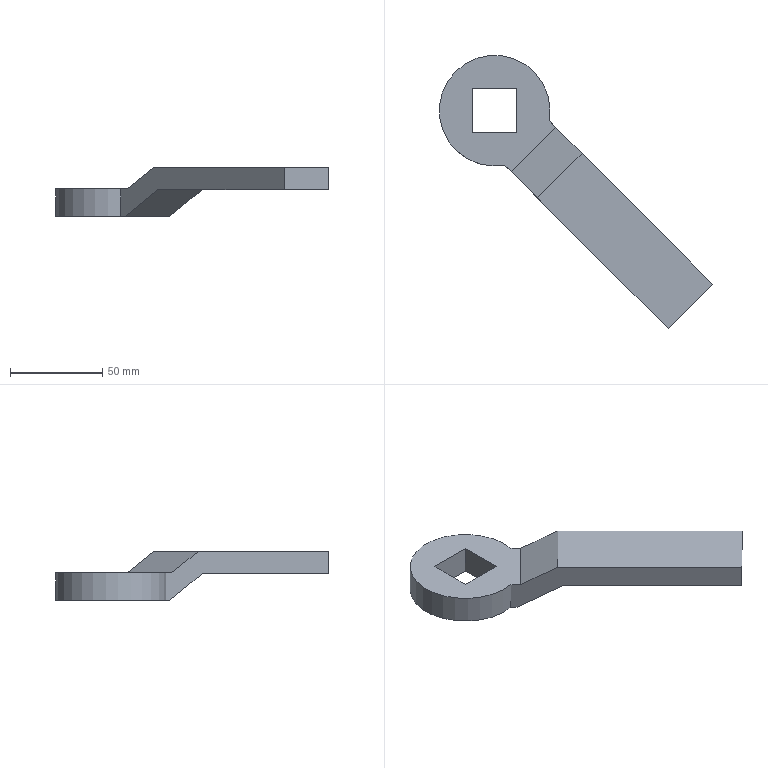Component | NX | WRENCH | 1 solid | 14 faces | box 148.09 x 148.09 x 26.55 mm | volume 84920 mm3 | plane 13 | cylinder 1 | commonest cylinder face diameters 60 x1
STEP:
#1=CARTESIAN_POINT('',(0.,0.,0.));
#2=DIRECTION('',(0.,0.,1.));
#3=DIRECTION('',(1.,0.,0.));
#4=AXIS2_PLACEMENT_3D('',#1,#2,#3);
#5=CARTESIAN_POINT('',(1.86,-30.695,193.134));
#6=VERTEX_POINT('',#5);
#7=CARTESIAN_POINT('',(25.901,-6.653,193.134));
#8=VERTEX_POINT('',#7);
#9=CARTESIAN_POINT('',(1.86,-30.695,193.134));
#10=DIRECTION('',(0.7071,0.7071,0.));
#11=VECTOR('',#10,1.);
#12=LINE('',#9,#11);
#13=CARTESIAN_POINT('',(1.86,-30.695,193.134));
#14=DIRECTION('',(-0.3536,0.3536,0.866));
#15=DIRECTION('',(0.6124,-0.6124,0.5));
#16=AXIS2_PLACEMENT_3D('',#13,#14,#15);
#17=PLANE('',#16);
#18=CARTESIAN_POINT('',(0.,0.));
#19=DIRECTION('',(-0.,1.));
#20=VECTOR('',#19,1.);
#21=LINE('',#18,#20);
#22=(GEOMETRIC_REPRESENTATION_CONTEXT(2)PARAMETRIC_REPRESENTATION_CONTEXT()REPRESENTATION_CONTEXT('',''));
#23=DEFINITIONAL_REPRESENTATION('',(#21),#22);
#24=PCURVE('',#17,#23);
#25=CARTESIAN_POINT('',(-5.932,1.139,193.134));
#26=DIRECTION('',(0.,0.,-1.));
#27=DIRECTION('',(-0.7071,0.7071,0.));
#28=AXIS2_PLACEMENT_3D('',#25,#26,#27);
#29=PLANE('',#28);
#30=CARTESIAN_POINT('',(-28.019,-17.));
#31=DIRECTION('',(0.,1.));
#32=VECTOR('',#31,1.);
#33=LINE('',#30,#32);
#34=(GEOMETRIC_REPRESENTATION_CONTEXT(2)PARAMETRIC_REPRESENTATION_CONTEXT()REPRESENTATION_CONTEXT('',''));
#35=DEFINITIONAL_REPRESENTATION('',(#33),#34);
#36=PCURVE('',#29,#35);
#37=SURFACE_CURVE('',#12,(#24,#36),.PCURVE_S1.);
#38=EDGE_CURVE('',#6,#8,#37,.T.);
#39=ORIENTED_EDGE('',*,*,#38,.T.);
#40=CARTESIAN_POINT('',(43.718,-24.469,207.681));
#41=VERTEX_POINT('',#40);
#42=CARTESIAN_POINT('',(25.901,-6.653,193.134));
#43=DIRECTION('',(0.6124,-0.6124,0.5));
#44=VECTOR('',#43,1.);
#45=LINE('',#42,#44);
#46=CARTESIAN_POINT('',(-0.,34.));
#47=DIRECTION('',(1.,0.));
#48=VECTOR('',#47,1.);
#49=LINE('',#46,#48);
#50=(GEOMETRIC_REPRESENTATION_CONTEXT(2)PARAMETRIC_REPRESENTATION_CONTEXT()REPRESENTATION_CONTEXT('',''));
#51=DEFINITIONAL_REPRESENTATION('',(#49),#50);
#52=PCURVE('',#17,#51);
#53=CARTESIAN_POINT('',(6.089,13.16,193.134));
#54=DIRECTION('',(-0.7071,-0.7071,0.));
#55=DIRECTION('',(0.,0.,-1.));
#56=AXIS2_PLACEMENT_3D('',#53,#54,#55);
#57=PLANE('',#56);
#58=CARTESIAN_POINT('',(0.,28.019));
#59=DIRECTION('',(-0.5,0.866));
#60=VECTOR('',#59,1.);
#61=LINE('',#58,#60);
#62=(GEOMETRIC_REPRESENTATION_CONTEXT(2)PARAMETRIC_REPRESENTATION_CONTEXT()REPRESENTATION_CONTEXT('',''));
#63=DEFINITIONAL_REPRESENTATION('',(#61),#62);
#64=PCURVE('',#57,#63);
#65=SURFACE_CURVE('',#45,(#52,#64),.PCURVE_S1.);
#66=EDGE_CURVE('',#8,#41,#65,.T.);
#67=ORIENTED_EDGE('',*,*,#66,.T.);
#68=CARTESIAN_POINT('',(19.676,-48.511,207.681));
#69=VERTEX_POINT('',#68);
#70=CARTESIAN_POINT('',(19.676,-48.511,207.681));
#71=DIRECTION('',(0.7071,0.7071,0.));
#72=VECTOR('',#71,1.);
#73=LINE('',#70,#72);
#74=CARTESIAN_POINT('',(29.094,0.));
#75=DIRECTION('',(-0.,1.));
#76=VECTOR('',#75,1.);
#77=LINE('',#74,#76);
#78=(GEOMETRIC_REPRESENTATION_CONTEXT(2)PARAMETRIC_REPRESENTATION_CONTEXT()REPRESENTATION_CONTEXT('',''));
#79=DEFINITIONAL_REPRESENTATION('',(#77),#78);
#80=PCURVE('',#17,#79);
#81=CARTESIAN_POINT('',(19.676,-48.511,207.681));
#82=DIRECTION('',(0.,0.,1.));
#83=DIRECTION('',(0.7071,-0.7071,0.));
#84=AXIS2_PLACEMENT_3D('',#81,#82,#83);
#85=PLANE('',#84);
#86=CARTESIAN_POINT('',(0.,0.));
#87=DIRECTION('',(0.,1.));
#88=VECTOR('',#87,1.);
#89=LINE('',#86,#88);
#90=(GEOMETRIC_REPRESENTATION_CONTEXT(2)PARAMETRIC_REPRESENTATION_CONTEXT()REPRESENTATION_CONTEXT('',''));
#91=DEFINITIONAL_REPRESENTATION('',(#89),#90);
#92=PCURVE('',#85,#91);
#93=SURFACE_CURVE('',#73,(#80,#92),.PCURVE_S1.);
#94=EDGE_CURVE('',#69,#41,#93,.T.);
#95=ORIENTED_EDGE('',*,*,#94,.F.);
#96=CARTESIAN_POINT('',(1.86,-30.695,193.134));
#97=DIRECTION('',(0.6124,-0.6124,0.5));
#98=VECTOR('',#97,1.);
#99=LINE('',#96,#98);
#100=CARTESIAN_POINT('',(0.,0.));
#101=DIRECTION('',(1.,0.));
#102=VECTOR('',#101,1.);
#103=LINE('',#100,#102);
#104=(GEOMETRIC_REPRESENTATION_CONTEXT(2)PARAMETRIC_REPRESENTATION_CONTEXT()REPRESENTATION_CONTEXT('',''));
#105=DEFINITIONAL_REPRESENTATION('',(#103),#104);
#106=PCURVE('',#17,#105);
#107=CARTESIAN_POINT('',(-17.953,-10.882,193.134));
#108=DIRECTION('',(-0.7071,-0.7071,0.));
#109=DIRECTION('',(0.,0.,-1.));
#110=AXIS2_PLACEMENT_3D('',#107,#108,#109);
#111=PLANE('',#110);
#112=CARTESIAN_POINT('',(0.,28.019));
#113=DIRECTION('',(-0.5,0.866));
#114=VECTOR('',#113,1.);
#115=LINE('',#112,#114);
#116=(GEOMETRIC_REPRESENTATION_CONTEXT(2)PARAMETRIC_REPRESENTATION_CONTEXT()REPRESENTATION_CONTEXT('',''));
#117=DEFINITIONAL_REPRESENTATION('',(#115),#116);
#118=PCURVE('',#111,#117);
#119=SURFACE_CURVE('',#99,(#106,#118),.PCURVE_S1.);
#120=EDGE_CURVE('',#6,#69,#119,.T.);
#121=ORIENTED_EDGE('',*,*,#120,.F.);
#122=EDGE_LOOP('',(#39,#67,#95,#121));
#123=FACE_BOUND('',#122,.T.);
#124=ADVANCED_FACE('',(#123),#17,.F.);
#125=CARTESIAN_POINT('',(-17.932,13.139,208.134));
#126=VERTEX_POINT('',#125);
#127=CARTESIAN_POINT('',(-17.932,-10.861,208.134));
#128=VERTEX_POINT('',#127);
#129=CARTESIAN_POINT('',(-17.932,13.139,208.134));
#130=DIRECTION('',(0.,-1.,0.));
#131=VECTOR('',#130,1.);
#132=LINE('',#129,#131);
#133=CARTESIAN_POINT('',(-5.932,1.139,208.134));
#134=DIRECTION('',(0.,0.,1.));
#135=DIRECTION('',(0.7071,-0.7071,0.));
#136=AXIS2_PLACEMENT_3D('',#133,#134,#135);
#137=PLANE('',#136);
#138=CARTESIAN_POINT('',(-16.971,0.));
#139=DIRECTION('',(0.7071,-0.7071));
#140=VECTOR('',#139,1.);
#141=LINE('',#138,#140);
#142=(GEOMETRIC_REPRESENTATION_CONTEXT(2)PARAMETRIC_REPRESENTATION_CONTEXT()REPRESENTATION_CONTEXT('',''));
#143=DEFINITIONAL_REPRESENTATION('',(#141),#142);
#144=PCURVE('',#137,#143);
#145=CARTESIAN_POINT('',(-17.932,13.139,191.134));
#146=DIRECTION('',(-1.,0.,0.));
#147=DIRECTION('',(0.,-1.,0.));
#148=AXIS2_PLACEMENT_3D('',#145,#146,#147);
#149=PLANE('',#148);
#150=CARTESIAN_POINT('',(0.,17.));
#151=DIRECTION('',(1.,0.));
#152=VECTOR('',#151,1.);
#153=LINE('',#150,#152);
#154=(GEOMETRIC_REPRESENTATION_CONTEXT(2)PARAMETRIC_REPRESENTATION_CONTEXT()REPRESENTATION_CONTEXT('',''));
#155=DEFINITIONAL_REPRESENTATION('',(#153),#154);
#156=PCURVE('',#149,#155);
#157=SURFACE_CURVE('',#132,(#144,#156),.PCURVE_S1.);
#158=EDGE_CURVE('',#126,#128,#157,.T.);
#159=ORIENTED_EDGE('',*,*,#158,.F.);
#160=CARTESIAN_POINT('',(6.068,13.139,208.134));
#161=VERTEX_POINT('',#160);
#162=CARTESIAN_POINT('',(6.068,13.139,208.134));
#163=DIRECTION('',(-1.,-0.,0.));
#164=VECTOR('',#163,1.);
#165=LINE('',#162,#164);
#166=CARTESIAN_POINT('',(-0.,16.971));
#167=DIRECTION('',(-0.7071,-0.7071));
#168=VECTOR('',#167,1.);
#169=LINE('',#166,#168);
#170=(GEOMETRIC_REPRESENTATION_CONTEXT(2)PARAMETRIC_REPRESENTATION_CONTEXT()REPRESENTATION_CONTEXT('',''));
#171=DEFINITIONAL_REPRESENTATION('',(#169),#170);
#172=PCURVE('',#137,#171);
#173=CARTESIAN_POINT('',(6.068,13.139,191.134));
#174=DIRECTION('',(-0.,1.,0.));
#175=DIRECTION('',(-1.,-0.,0.));
#176=AXIS2_PLACEMENT_3D('',#173,#174,#175);
#177=PLANE('',#176);
#178=CARTESIAN_POINT('',(0.,17.));
#179=DIRECTION('',(1.,0.));
#180=VECTOR('',#179,1.);
#181=LINE('',#178,#180);
#182=(GEOMETRIC_REPRESENTATION_CONTEXT(2)PARAMETRIC_REPRESENTATION_CONTEXT()REPRESENTATION_CONTEXT('',''));
#183=DEFINITIONAL_REPRESENTATION('',(#181),#182);
#184=PCURVE('',#177,#183);
#185=SURFACE_CURVE('',#165,(#172,#184),.PCURVE_S1.);
#186=EDGE_CURVE('',#161,#126,#185,.T.);
#187=ORIENTED_EDGE('',*,*,#186,.F.);
#188=CARTESIAN_POINT('',(6.068,-10.861,208.134));
#189=VERTEX_POINT('',#188);
#190=CARTESIAN_POINT('',(6.068,-10.861,208.134));
#191=DIRECTION('',(-0.,1.,0.));
#192=VECTOR('',#191,1.);
#193=LINE('',#190,#192);
#194=CARTESIAN_POINT('',(16.971,0.));
#195=DIRECTION('',(-0.7071,0.7071));
#196=VECTOR('',#195,1.);
#197=LINE('',#194,#196);
#198=(GEOMETRIC_REPRESENTATION_CONTEXT(2)PARAMETRIC_REPRESENTATION_CONTEXT()REPRESENTATION_CONTEXT('',''));
#199=DEFINITIONAL_REPRESENTATION('',(#197),#198);
#200=PCURVE('',#137,#199);
#201=CARTESIAN_POINT('',(6.068,-10.861,191.134));
#202=DIRECTION('',(1.,0.,0.));
#203=DIRECTION('',(-0.,1.,0.));
#204=AXIS2_PLACEMENT_3D('',#201,#202,#203);
#205=PLANE('',#204);
#206=CARTESIAN_POINT('',(0.,17.));
#207=DIRECTION('',(1.,0.));
#208=VECTOR('',#207,1.);
#209=LINE('',#206,#208);
#210=(GEOMETRIC_REPRESENTATION_CONTEXT(2)PARAMETRIC_REPRESENTATION_CONTEXT()REPRESENTATION_CONTEXT('',''));
#211=DEFINITIONAL_REPRESENTATION('',(#209),#210);
#212=PCURVE('',#205,#211);
#213=SURFACE_CURVE('',#193,(#200,#212),.PCURVE_S1.);
#214=EDGE_CURVE('',#189,#161,#213,.T.);
#215=ORIENTED_EDGE('',*,*,#214,.F.);
#216=CARTESIAN_POINT('',(-17.932,-10.861,208.134));
#217=DIRECTION('',(1.,0.,0.));
#218=VECTOR('',#217,1.);
#219=LINE('',#216,#218);
#220=CARTESIAN_POINT('',(0.,-16.971));
#221=DIRECTION('',(0.7071,0.7071));
#222=VECTOR('',#221,1.);
#223=LINE('',#220,#222);
#224=(GEOMETRIC_REPRESENTATION_CONTEXT(2)PARAMETRIC_REPRESENTATION_CONTEXT()REPRESENTATION_CONTEXT('',''));
#225=DEFINITIONAL_REPRESENTATION('',(#223),#224);
#226=PCURVE('',#137,#225);
#227=CARTESIAN_POINT('',(-17.932,-10.861,191.134));
#228=DIRECTION('',(0.,-1.,0.));
#229=DIRECTION('',(1.,0.,0.));
#230=AXIS2_PLACEMENT_3D('',#227,#228,#229);
#231=PLANE('',#230);
#232=CARTESIAN_POINT('',(0.,17.));
#233=DIRECTION('',(1.,0.));
#234=VECTOR('',#233,1.);
#235=LINE('',#232,#234);
#236=(GEOMETRIC_REPRESENTATION_CONTEXT(2)PARAMETRIC_REPRESENTATION_CONTEXT()REPRESENTATION_CONTEXT('',''));
#237=DEFINITIONAL_REPRESENTATION('',(#235),#236);
#238=PCURVE('',#231,#237);
#239=SURFACE_CURVE('',#219,(#226,#238),.PCURVE_S1.);
#240=EDGE_CURVE('',#128,#189,#239,.T.);
#241=ORIENTED_EDGE('',*,*,#240,.F.);
#242=EDGE_LOOP('',(#159,#187,#215,#241));
#243=FACE_BOUND('',#242,.T.);
#244=CARTESIAN_POINT('',(-0.4744,-28.361,208.134));
#245=VERTEX_POINT('',#244);
#246=CARTESIAN_POINT('',(23.567,-4.319,208.134));
#247=VERTEX_POINT('',#246);
#248=CARTESIAN_POINT('',(-5.932,1.139,208.134));
#249=DIRECTION('',(0.,0.,-1.));
#250=DIRECTION('',(0.7071,-0.7071,0.));
#251=AXIS2_PLACEMENT_3D('',#248,#249,#250);
#252=CIRCLE('',#251,30.);
#253=CARTESIAN_POINT('',(30.,0.));
#254=CARTESIAN_POINT('',(30.,-51.962));
#255=CARTESIAN_POINT('',(-15.,-25.981));
#256=CARTESIAN_POINT('',(-60.,-0.));
#257=CARTESIAN_POINT('',(-15.,25.981));
#258=CARTESIAN_POINT('',(30.,51.962));
#259=CARTESIAN_POINT('',(30.,0.));
#260=(BOUNDED_CURVE()B_SPLINE_CURVE(2,(#253,#254,#255,#256,#257,#258,#259),.UNSPECIFIED.,.T.,.F.)B_SPLINE_CURVE_WITH_KNOTS((1,2,2,2,2,1),(-2.094,0.,2.094,4.189,6.283,8.378),.UNSPECIFIED.)CURVE()GEOMETRIC_REPRESENTATION_ITEM()RATIONAL_B_SPLINE_CURVE((1.,0.5,1.,0.5,1.,0.5,1.))REPRESENTATION_ITEM(''));
#261=(GEOMETRIC_REPRESENTATION_CONTEXT(2)PARAMETRIC_REPRESENTATION_CONTEXT()REPRESENTATION_CONTEXT('',''));
#262=DEFINITIONAL_REPRESENTATION('',(#260),#261);
#263=PCURVE('',#137,#262);
#264=CARTESIAN_POINT('',(-5.932,1.139,193.134));
#265=DIRECTION('',(0.,0.,1.));
#266=DIRECTION('',(0.7071,-0.7071,0.));
#267=AXIS2_PLACEMENT_3D('',#264,#265,#266);
#268=CYLINDRICAL_SURFACE('',#267,30.);
#269=CARTESIAN_POINT('',(6.283,15.));
#270=DIRECTION('',(-1.,0.));
#271=VECTOR('',#270,1.);
#272=LINE('',#269,#271);
#273=(GEOMETRIC_REPRESENTATION_CONTEXT(2)PARAMETRIC_REPRESENTATION_CONTEXT()REPRESENTATION_CONTEXT('',''));
#274=DEFINITIONAL_REPRESENTATION('',(#272),#273);
#275=PCURVE('',#268,#274);
#276=SURFACE_CURVE('',#252,(#263,#275),.PCURVE_S1.);
#277=EDGE_CURVE('',#245,#247,#276,.T.);
#278=ORIENTED_EDGE('',*,*,#277,.F.);
#279=CARTESIAN_POINT('',(3.26,-32.095,208.134));
#280=VERTEX_POINT('',#279);
#281=CARTESIAN_POINT('',(-17.953,-10.882,208.134));
#282=DIRECTION('',(-0.7071,0.7071,0.));
#283=VECTOR('',#282,1.);
#284=LINE('',#281,#283);
#285=CARTESIAN_POINT('',(0.,-17.));
#286=DIRECTION('',(-1.,0.));
#287=VECTOR('',#286,1.);
#288=LINE('',#285,#287);
#289=(GEOMETRIC_REPRESENTATION_CONTEXT(2)PARAMETRIC_REPRESENTATION_CONTEXT()REPRESENTATION_CONTEXT('',''));
#290=DEFINITIONAL_REPRESENTATION('',(#288),#289);
#291=PCURVE('',#137,#290);
#292=CARTESIAN_POINT('',(-15.,0.));
#293=DIRECTION('',(0.,-1.));
#294=VECTOR('',#293,1.);
#295=LINE('',#292,#294);
#296=(GEOMETRIC_REPRESENTATION_CONTEXT(2)PARAMETRIC_REPRESENTATION_CONTEXT()REPRESENTATION_CONTEXT('',''));
#297=DEFINITIONAL_REPRESENTATION('',(#295),#296);
#298=PCURVE('',#111,#297);
#299=SURFACE_CURVE('',#284,(#291,#298),.PCURVE_S1.);
#300=EDGE_CURVE('',#280,#245,#299,.T.);
#301=ORIENTED_EDGE('',*,*,#300,.F.);
#302=CARTESIAN_POINT('',(27.302,-8.054,208.134));
#303=VERTEX_POINT('',#302);
#304=CARTESIAN_POINT('',(15.281,-20.074,208.134));
#305=DIRECTION('',(0.7071,0.7071,0.));
#306=VECTOR('',#305,1.);
#307=LINE('',#304,#306);
#308=CARTESIAN_POINT('',(30.,0.));
#309=DIRECTION('',(0.,1.));
#310=VECTOR('',#309,1.);
#311=LINE('',#308,#310);
#312=(GEOMETRIC_REPRESENTATION_CONTEXT(2)PARAMETRIC_REPRESENTATION_CONTEXT()REPRESENTATION_CONTEXT('',''));
#313=DEFINITIONAL_REPRESENTATION('',(#311),#312);
#314=PCURVE('',#137,#313);
#315=CARTESIAN_POINT('',(17.402,-46.237,219.681));
#316=DIRECTION('',(0.3536,-0.3536,-0.866));
#317=DIRECTION('',(-0.6124,0.6124,-0.5));
#318=AXIS2_PLACEMENT_3D('',#315,#316,#317);
#319=PLANE('',#318);
#320=CARTESIAN_POINT('',(23.094,17.));
#321=DIRECTION('',(0.,1.));
#322=VECTOR('',#321,1.);
#323=LINE('',#320,#322);
#324=(GEOMETRIC_REPRESENTATION_CONTEXT(2)PARAMETRIC_REPRESENTATION_CONTEXT()REPRESENTATION_CONTEXT('',''));
#325=DEFINITIONAL_REPRESENTATION('',(#323),#324);
#326=PCURVE('',#319,#325);
#327=SURFACE_CURVE('',#307,(#314,#326),.PCURVE_S1.);
#328=EDGE_CURVE('',#280,#303,#327,.T.);
#329=ORIENTED_EDGE('',*,*,#328,.T.);
#330=CARTESIAN_POINT('',(6.089,13.16,208.134));
#331=DIRECTION('',(-0.7071,0.7071,0.));
#332=VECTOR('',#331,1.);
#333=LINE('',#330,#332);
#334=CARTESIAN_POINT('',(-0.,17.));
#335=DIRECTION('',(-1.,0.));
#336=VECTOR('',#335,1.);
#337=LINE('',#334,#336);
#338=(GEOMETRIC_REPRESENTATION_CONTEXT(2)PARAMETRIC_REPRESENTATION_CONTEXT()REPRESENTATION_CONTEXT('',''));
#339=DEFINITIONAL_REPRESENTATION('',(#337),#338);
#340=PCURVE('',#137,#339);
#341=CARTESIAN_POINT('',(-15.,0.));
#342=DIRECTION('',(0.,-1.));
#343=VECTOR('',#342,1.);
#344=LINE('',#341,#343);
#345=(GEOMETRIC_REPRESENTATION_CONTEXT(2)PARAMETRIC_REPRESENTATION_CONTEXT()REPRESENTATION_CONTEXT('',''));
#346=DEFINITIONAL_REPRESENTATION('',(#344),#345);
#347=PCURVE('',#57,#346);
#348=SURFACE_CURVE('',#333,(#340,#347),.PCURVE_S1.);
#349=EDGE_CURVE('',#303,#247,#348,.T.);
#350=ORIENTED_EDGE('',*,*,#349,.T.);
#351=EDGE_LOOP('',(#278,#301,#329,#350));
#352=FACE_BOUND('',#351,.T.);
#353=ADVANCED_FACE('',(#243,#352),#137,.T.);
#354=CARTESIAN_POINT('',(-17.932,-10.861,193.134));
#355=VERTEX_POINT('',#354);
#356=CARTESIAN_POINT('',(-17.932,13.139,193.134));
#357=VERTEX_POINT('',#356);
#358=CARTESIAN_POINT('',(-17.932,1.139,193.134));
#359=DIRECTION('',(0.,1.,0.));
#360=VECTOR('',#359,1.);
#361=LINE('',#358,#360);
#362=CARTESIAN_POINT('',(8.485,-8.485));
#363=DIRECTION('',(0.7071,0.7071));
#364=VECTOR('',#363,1.);
#365=LINE('',#362,#364);
#366=(GEOMETRIC_REPRESENTATION_CONTEXT(2)PARAMETRIC_REPRESENTATION_CONTEXT()REPRESENTATION_CONTEXT('',''));
#367=DEFINITIONAL_REPRESENTATION('',(#365),#366);
#368=PCURVE('',#29,#367);
#369=CARTESIAN_POINT('',(12.,2.));
#370=DIRECTION('',(-1.,0.));
#371=VECTOR('',#370,1.);
#372=LINE('',#369,#371);
#373=(GEOMETRIC_REPRESENTATION_CONTEXT(2)PARAMETRIC_REPRESENTATION_CONTEXT()REPRESENTATION_CONTEXT('',''));
#374=DEFINITIONAL_REPRESENTATION('',(#372),#373);
#375=PCURVE('',#149,#374);
#376=SURFACE_CURVE('',#361,(#368,#375),.PCURVE_S1.);
#377=EDGE_CURVE('',#355,#357,#376,.T.);
#378=ORIENTED_EDGE('',*,*,#377,.F.);
#379=CARTESIAN_POINT('',(6.068,-10.861,193.134));
#380=VERTEX_POINT('',#379);
#381=CARTESIAN_POINT('',(-5.932,-10.861,193.134));
#382=DIRECTION('',(-1.,-0.,0.));
#383=VECTOR('',#382,1.);
#384=LINE('',#381,#383);
#385=CARTESIAN_POINT('',(-8.485,-8.485));
#386=DIRECTION('',(0.7071,-0.7071));
#387=VECTOR('',#386,1.);
#388=LINE('',#385,#387);
#389=(GEOMETRIC_REPRESENTATION_CONTEXT(2)PARAMETRIC_REPRESENTATION_CONTEXT()REPRESENTATION_CONTEXT('',''));
#390=DEFINITIONAL_REPRESENTATION('',(#388),#389);
#391=PCURVE('',#29,#390);
#392=CARTESIAN_POINT('',(12.,2.));
#393=DIRECTION('',(-1.,0.));
#394=VECTOR('',#393,1.);
#395=LINE('',#392,#394);
#396=(GEOMETRIC_REPRESENTATION_CONTEXT(2)PARAMETRIC_REPRESENTATION_CONTEXT()REPRESENTATION_CONTEXT('',''));
#397=DEFINITIONAL_REPRESENTATION('',(#395),#396);
#398=PCURVE('',#231,#397);
#399=SURFACE_CURVE('',#384,(#391,#398),.PCURVE_S1.);
#400=EDGE_CURVE('',#380,#355,#399,.T.);
#401=ORIENTED_EDGE('',*,*,#400,.F.);
#402=CARTESIAN_POINT('',(6.068,13.139,193.134));
#403=VERTEX_POINT('',#402);
#404=CARTESIAN_POINT('',(6.068,1.139,193.134));
#405=DIRECTION('',(0.,-1.,0.));
#406=VECTOR('',#405,1.);
#407=LINE('',#404,#406);
#408=CARTESIAN_POINT('',(-8.485,8.485));
#409=DIRECTION('',(-0.7071,-0.7071));
#410=VECTOR('',#409,1.);
#411=LINE('',#408,#410);
#412=(GEOMETRIC_REPRESENTATION_CONTEXT(2)PARAMETRIC_REPRESENTATION_CONTEXT()REPRESENTATION_CONTEXT('',''));
#413=DEFINITIONAL_REPRESENTATION('',(#411),#412);
#414=PCURVE('',#29,#413);
#415=CARTESIAN_POINT('',(12.,2.));
#416=DIRECTION('',(-1.,0.));
#417=VECTOR('',#416,1.);
#418=LINE('',#415,#417);
#419=(GEOMETRIC_REPRESENTATION_CONTEXT(2)PARAMETRIC_REPRESENTATION_CONTEXT()REPRESENTATION_CONTEXT('',''));
#420=DEFINITIONAL_REPRESENTATION('',(#418),#419);
#421=PCURVE('',#205,#420);
#422=SURFACE_CURVE('',#407,(#414,#421),.PCURVE_S1.);
#423=EDGE_CURVE('',#403,#380,#422,.T.);
#424=ORIENTED_EDGE('',*,*,#423,.F.);
#425=CARTESIAN_POINT('',(-5.932,13.139,193.134));
#426=DIRECTION('',(1.,0.,0.));
#427=VECTOR('',#426,1.);
#428=LINE('',#425,#427);
#429=CARTESIAN_POINT('',(8.485,8.485));
#430=DIRECTION('',(-0.7071,0.7071));
#431=VECTOR('',#430,1.);
#432=LINE('',#429,#431);
#433=(GEOMETRIC_REPRESENTATION_CONTEXT(2)PARAMETRIC_REPRESENTATION_CONTEXT()REPRESENTATION_CONTEXT('',''));
#434=DEFINITIONAL_REPRESENTATION('',(#432),#433);
#435=PCURVE('',#29,#434);
#436=CARTESIAN_POINT('',(12.,2.));
#437=DIRECTION('',(-1.,0.));
#438=VECTOR('',#437,1.);
#439=LINE('',#436,#438);
#440=(GEOMETRIC_REPRESENTATION_CONTEXT(2)PARAMETRIC_REPRESENTATION_CONTEXT()REPRESENTATION_CONTEXT('',''));
#441=DEFINITIONAL_REPRESENTATION('',(#439),#440);
#442=PCURVE('',#177,#441);
#443=SURFACE_CURVE('',#428,(#435,#442),.PCURVE_S1.);
#444=EDGE_CURVE('',#357,#403,#443,.T.);
#445=ORIENTED_EDGE('',*,*,#444,.F.);
#446=EDGE_LOOP('',(#378,#401,#424,#445));
#447=FACE_BOUND('',#446,.T.);
#448=CARTESIAN_POINT('',(23.567,-4.319,193.134));
#449=VERTEX_POINT('',#448);
#450=CARTESIAN_POINT('',(-0.4744,-28.361,193.134));
#451=VERTEX_POINT('',#450);
#452=CARTESIAN_POINT('',(-5.932,1.139,193.134));
#453=DIRECTION('',(0.,0.,1.));
#454=DIRECTION('',(0.7071,-0.7071,0.));
#455=AXIS2_PLACEMENT_3D('',#452,#453,#454);
#456=CIRCLE('',#455,30.);
#457=CARTESIAN_POINT('',(-30.,0.));
#458=CARTESIAN_POINT('',(-30.,51.962));
#459=CARTESIAN_POINT('',(15.,25.981));
#460=CARTESIAN_POINT('',(60.,0.));
#461=CARTESIAN_POINT('',(15.,-25.981));
#462=CARTESIAN_POINT('',(-30.,-51.962));
#463=CARTESIAN_POINT('',(-30.,0.));
#464=(BOUNDED_CURVE()B_SPLINE_CURVE(2,(#457,#458,#459,#460,#461,#462,#463),.UNSPECIFIED.,.T.,.F.)B_SPLINE_CURVE_WITH_KNOTS((1,2,2,2,2,1),(-2.094,0.,2.094,4.189,6.283,8.378),.UNSPECIFIED.)CURVE()GEOMETRIC_REPRESENTATION_ITEM()RATIONAL_B_SPLINE_CURVE((1.,0.5,1.,0.5,1.,0.5,1.))REPRESENTATION_ITEM(''));
#465=(GEOMETRIC_REPRESENTATION_CONTEXT(2)PARAMETRIC_REPRESENTATION_CONTEXT()REPRESENTATION_CONTEXT('',''));
#466=DEFINITIONAL_REPRESENTATION('',(#464),#465);
#467=PCURVE('',#29,#466);
#468=CARTESIAN_POINT('',(0.,0.));
#469=DIRECTION('',(1.,0.));
#470=VECTOR('',#469,1.);
#471=LINE('',#468,#470);
#472=(GEOMETRIC_REPRESENTATION_CONTEXT(2)PARAMETRIC_REPRESENTATION_CONTEXT()REPRESENTATION_CONTEXT('',''));
#473=DEFINITIONAL_REPRESENTATION('',(#471),#472);
#474=PCURVE('',#268,#473);
#475=SURFACE_CURVE('',#456,(#467,#474),.PCURVE_S1.);
#476=EDGE_CURVE('',#449,#451,#475,.T.);
#477=ORIENTED_EDGE('',*,*,#476,.F.);
#478=CARTESIAN_POINT('',(18.802,0.4465,193.134));
#479=DIRECTION('',(0.7071,-0.7071,0.));
#480=VECTOR('',#479,1.);
#481=LINE('',#478,#480);
#482=CARTESIAN_POINT('',(-17.979,17.));
#483=DIRECTION('',(-1.,0.));
#484=VECTOR('',#483,1.);
#485=LINE('',#482,#484);
#486=(GEOMETRIC_REPRESENTATION_CONTEXT(2)PARAMETRIC_REPRESENTATION_CONTEXT()REPRESENTATION_CONTEXT('',''));
#487=DEFINITIONAL_REPRESENTATION('',(#485),#486);
#488=PCURVE('',#29,#487);
#489=CARTESIAN_POINT('',(0.,17.979));
#490=DIRECTION('',(-0.,1.));
#491=VECTOR('',#490,1.);
#492=LINE('',#489,#491);
#493=(GEOMETRIC_REPRESENTATION_CONTEXT(2)PARAMETRIC_REPRESENTATION_CONTEXT()REPRESENTATION_CONTEXT('',''));
#494=DEFINITIONAL_REPRESENTATION('',(#492),#493);
#495=PCURVE('',#57,#494);
#496=SURFACE_CURVE('',#481,(#488,#495),.PCURVE_S1.);
#497=EDGE_CURVE('',#449,#8,#496,.T.);
#498=ORIENTED_EDGE('',*,*,#497,.T.);
#499=ORIENTED_EDGE('',*,*,#38,.F.);
#500=CARTESIAN_POINT('',(-5.24,-23.595,193.134));
#501=DIRECTION('',(0.7071,-0.7071,0.));
#502=VECTOR('',#501,1.);
#503=LINE('',#500,#502);
#504=CARTESIAN_POINT('',(-17.979,-17.));
#505=DIRECTION('',(-1.,0.));
#506=VECTOR('',#505,1.);
#507=LINE('',#504,#506);
#508=(GEOMETRIC_REPRESENTATION_CONTEXT(2)PARAMETRIC_REPRESENTATION_CONTEXT()REPRESENTATION_CONTEXT('',''));
#509=DEFINITIONAL_REPRESENTATION('',(#507),#508);
#510=PCURVE('',#29,#509);
#511=CARTESIAN_POINT('',(0.,17.979));
#512=DIRECTION('',(-0.,1.));
#513=VECTOR('',#512,1.);
#514=LINE('',#511,#513);
#515=(GEOMETRIC_REPRESENTATION_CONTEXT(2)PARAMETRIC_REPRESENTATION_CONTEXT()REPRESENTATION_CONTEXT('',''));
#516=DEFINITIONAL_REPRESENTATION('',(#514),#515);
#517=PCURVE('',#111,#516);
#518=SURFACE_CURVE('',#503,(#510,#517),.PCURVE_S1.);
#519=EDGE_CURVE('',#451,#6,#518,.T.);
#520=ORIENTED_EDGE('',*,*,#519,.F.);
#521=EDGE_LOOP('',(#477,#498,#499,#520));
#522=FACE_BOUND('',#521,.T.);
#523=ADVANCED_FACE('',(#447,#522),#29,.T.);
#524=CARTESIAN_POINT('',(-0.4744,-28.361,193.134));
#525=DIRECTION('',(0.,0.,-1.));
#526=VECTOR('',#525,1.);
#527=LINE('',#524,#526);
#528=CARTESIAN_POINT('',(5.681,0.));
#529=DIRECTION('',(0.,-1.));
#530=VECTOR('',#529,1.);
#531=LINE('',#528,#530);
#532=(GEOMETRIC_REPRESENTATION_CONTEXT(2)PARAMETRIC_REPRESENTATION_CONTEXT()REPRESENTATION_CONTEXT('',''));
#533=DEFINITIONAL_REPRESENTATION('',(#531),#532);
#534=PCURVE('',#268,#533);
#535=CARTESIAN_POINT('',(0.,24.718));
#536=DIRECTION('',(1.,0.));
#537=VECTOR('',#536,1.);
#538=LINE('',#535,#537);
#539=(GEOMETRIC_REPRESENTATION_CONTEXT(2)PARAMETRIC_REPRESENTATION_CONTEXT()REPRESENTATION_CONTEXT('',''));
#540=DEFINITIONAL_REPRESENTATION('',(#538),#539);
#541=PCURVE('',#111,#540);
#542=SURFACE_CURVE('',#527,(#534,#541),.PCURVE_S1.);
#543=EDGE_CURVE('',#245,#451,#542,.T.);
#544=ORIENTED_EDGE('',*,*,#543,.F.);
#545=ORIENTED_EDGE('',*,*,#277,.T.);
#546=CARTESIAN_POINT('',(23.567,-4.319,193.134));
#547=DIRECTION('',(0.,0.,-1.));
#548=VECTOR('',#547,1.);
#549=LINE('',#546,#548);
#550=CARTESIAN_POINT('',(0.6025,0.));
#551=DIRECTION('',(0.,-1.));
#552=VECTOR('',#551,1.);
#553=LINE('',#550,#552);
#554=(GEOMETRIC_REPRESENTATION_CONTEXT(2)PARAMETRIC_REPRESENTATION_CONTEXT()REPRESENTATION_CONTEXT('',''));
#555=DEFINITIONAL_REPRESENTATION('',(#553),#554);
#556=PCURVE('',#268,#555);
#557=CARTESIAN_POINT('',(0.,24.718));
#558=DIRECTION('',(1.,0.));
#559=VECTOR('',#558,1.);
#560=LINE('',#557,#559);
#561=(GEOMETRIC_REPRESENTATION_CONTEXT(2)PARAMETRIC_REPRESENTATION_CONTEXT()REPRESENTATION_CONTEXT('',''));
#562=DEFINITIONAL_REPRESENTATION('',(#560),#561);
#563=PCURVE('',#57,#562);
#564=SURFACE_CURVE('',#549,(#556,#563),.PCURVE_S1.);
#565=EDGE_CURVE('',#247,#449,#564,.T.);
#566=ORIENTED_EDGE('',*,*,#565,.T.);
#567=ORIENTED_EDGE('',*,*,#476,.T.);
#568=EDGE_LOOP('',(#544,#545,#566,#567));
#569=FACE_BOUND('',#568,.T.);
#570=ADVANCED_FACE('',(#569),#268,.T.);
#571=CARTESIAN_POINT('',(112.155,-92.906,207.681));
#572=VERTEX_POINT('',#571);
#573=CARTESIAN_POINT('',(43.718,-24.469,207.681));
#574=DIRECTION('',(0.7071,-0.7071,0.));
#575=VECTOR('',#574,1.);
#576=LINE('',#573,#575);
#577=CARTESIAN_POINT('',(-0.,34.));
#578=DIRECTION('',(1.,0.));
#579=VECTOR('',#578,1.);
#580=LINE('',#577,#579);
#581=(GEOMETRIC_REPRESENTATION_CONTEXT(2)PARAMETRIC_REPRESENTATION_CONTEXT()REPRESENTATION_CONTEXT('',''));
#582=DEFINITIONAL_REPRESENTATION('',(#580),#581);
#583=PCURVE('',#85,#582);
#584=CARTESIAN_POINT('',(-14.547,53.215));
#585=DIRECTION('',(0.,1.));
#586=VECTOR('',#585,1.);
#587=LINE('',#584,#586);
#588=(GEOMETRIC_REPRESENTATION_CONTEXT(2)PARAMETRIC_REPRESENTATION_CONTEXT()REPRESENTATION_CONTEXT('',''));
#589=DEFINITIONAL_REPRESENTATION('',(#587),#588);
#590=PCURVE('',#57,#589);
#591=SURFACE_CURVE('',#576,(#583,#590),.PCURVE_S1.);
#592=EDGE_CURVE('',#41,#572,#591,.T.);
#593=ORIENTED_EDGE('',*,*,#592,.T.);
#594=CARTESIAN_POINT('',(88.113,-116.948,207.681));
#595=VERTEX_POINT('',#594);
#596=CARTESIAN_POINT('',(88.113,-116.948,207.681));
#597=DIRECTION('',(0.7071,0.7071,0.));
#598=VECTOR('',#597,1.);
#599=LINE('',#596,#598);
#600=CARTESIAN_POINT('',(96.785,0.));
#601=DIRECTION('',(0.,1.));
#602=VECTOR('',#601,1.);
#603=LINE('',#600,#602);
#604=(GEOMETRIC_REPRESENTATION_CONTEXT(2)PARAMETRIC_REPRESENTATION_CONTEXT()REPRESENTATION_CONTEXT('',''));
#605=DEFINITIONAL_REPRESENTATION('',(#603),#604);
#606=PCURVE('',#85,#605);
#607=CARTESIAN_POINT('',(88.113,-116.948,207.681));
#608=DIRECTION('',(-0.7071,0.7071,0.));
#609=DIRECTION('',(0.,0.,1.));
#610=AXIS2_PLACEMENT_3D('',#607,#608,#609);
#611=PLANE('',#610);
#612=CARTESIAN_POINT('',(0.,0.));
#613=DIRECTION('',(0.,1.));
#614=VECTOR('',#613,1.);
#615=LINE('',#612,#614);
#616=(GEOMETRIC_REPRESENTATION_CONTEXT(2)PARAMETRIC_REPRESENTATION_CONTEXT()REPRESENTATION_CONTEXT('',''));
#617=DEFINITIONAL_REPRESENTATION('',(#615),#616);
#618=PCURVE('',#611,#617);
#619=SURFACE_CURVE('',#599,(#606,#618),.PCURVE_S1.);
#620=EDGE_CURVE('',#595,#572,#619,.T.);
#621=ORIENTED_EDGE('',*,*,#620,.F.);
#622=CARTESIAN_POINT('',(19.676,-48.511,207.681));
#623=DIRECTION('',(0.7071,-0.7071,0.));
#624=VECTOR('',#623,1.);
#625=LINE('',#622,#624);
#626=CARTESIAN_POINT('',(0.,0.));
#627=DIRECTION('',(1.,0.));
#628=VECTOR('',#627,1.);
#629=LINE('',#626,#628);
#630=(GEOMETRIC_REPRESENTATION_CONTEXT(2)PARAMETRIC_REPRESENTATION_CONTEXT()REPRESENTATION_CONTEXT('',''));
#631=DEFINITIONAL_REPRESENTATION('',(#629),#630);
#632=PCURVE('',#85,#631);
#633=CARTESIAN_POINT('',(-14.547,53.215));
#634=DIRECTION('',(0.,1.));
#635=VECTOR('',#634,1.);
#636=LINE('',#633,#635);
#637=(GEOMETRIC_REPRESENTATION_CONTEXT(2)PARAMETRIC_REPRESENTATION_CONTEXT()REPRESENTATION_CONTEXT('',''));
#638=DEFINITIONAL_REPRESENTATION('',(#636),#637);
#639=PCURVE('',#111,#638);
#640=SURFACE_CURVE('',#625,(#632,#639),.PCURVE_S1.);
#641=EDGE_CURVE('',#69,#595,#640,.T.);
#642=ORIENTED_EDGE('',*,*,#641,.F.);
#643=ORIENTED_EDGE('',*,*,#94,.T.);
#644=EDGE_LOOP('',(#593,#621,#642,#643));
#645=FACE_BOUND('',#644,.T.);
#646=ADVANCED_FACE('',(#645),#85,.F.);
#647=CARTESIAN_POINT('',(112.155,-92.906,219.681));
#648=VERTEX_POINT('',#647);
#649=CARTESIAN_POINT('',(112.155,-92.906,207.681));
#650=DIRECTION('',(0.,0.,1.));
#651=VECTOR('',#650,1.);
#652=LINE('',#649,#651);
#653=CARTESIAN_POINT('',(0.,34.));
#654=DIRECTION('',(1.,0.));
#655=VECTOR('',#654,1.);
#656=LINE('',#653,#655);
#657=(GEOMETRIC_REPRESENTATION_CONTEXT(2)PARAMETRIC_REPRESENTATION_CONTEXT()REPRESENTATION_CONTEXT('',''));
#658=DEFINITIONAL_REPRESENTATION('',(#656),#657);
#659=PCURVE('',#611,#658);
#660=CARTESIAN_POINT('',(-14.547,150.));
#661=DIRECTION('',(-1.,0.));
#662=VECTOR('',#661,1.);
#663=LINE('',#660,#662);
#664=(GEOMETRIC_REPRESENTATION_CONTEXT(2)PARAMETRIC_REPRESENTATION_CONTEXT()REPRESENTATION_CONTEXT('',''));
#665=DEFINITIONAL_REPRESENTATION('',(#663),#664);
#666=PCURVE('',#57,#665);
#667=SURFACE_CURVE('',#652,(#659,#666),.PCURVE_S1.);
#668=EDGE_CURVE('',#572,#648,#667,.T.);
#669=ORIENTED_EDGE('',*,*,#668,.T.);
#670=CARTESIAN_POINT('',(88.113,-116.948,219.681));
#671=VERTEX_POINT('',#670);
#672=CARTESIAN_POINT('',(88.113,-116.948,219.681));
#673=DIRECTION('',(0.7071,0.7071,0.));
#674=VECTOR('',#673,1.);
#675=LINE('',#672,#674);
#676=CARTESIAN_POINT('',(12.,0.));
#677=DIRECTION('',(0.,1.));
#678=VECTOR('',#677,1.);
#679=LINE('',#676,#678);
#680=(GEOMETRIC_REPRESENTATION_CONTEXT(2)PARAMETRIC_REPRESENTATION_CONTEXT()REPRESENTATION_CONTEXT('',''));
#681=DEFINITIONAL_REPRESENTATION('',(#679),#680);
#682=PCURVE('',#611,#681);
#683=CARTESIAN_POINT('',(88.113,-116.948,219.681));
#684=DIRECTION('',(0.,0.,-1.));
#685=DIRECTION('',(-0.7071,0.7071,0.));
#686=AXIS2_PLACEMENT_3D('',#683,#684,#685);
#687=PLANE('',#686);
#688=CARTESIAN_POINT('',(0.,0.));
#689=DIRECTION('',(0.,1.));
#690=VECTOR('',#689,1.);
#691=LINE('',#688,#690);
#692=(GEOMETRIC_REPRESENTATION_CONTEXT(2)PARAMETRIC_REPRESENTATION_CONTEXT()REPRESENTATION_CONTEXT('',''));
#693=DEFINITIONAL_REPRESENTATION('',(#691),#692);
#694=PCURVE('',#687,#693);
#695=SURFACE_CURVE('',#675,(#682,#694),.PCURVE_S1.);
#696=EDGE_CURVE('',#671,#648,#695,.T.);
#697=ORIENTED_EDGE('',*,*,#696,.F.);
#698=CARTESIAN_POINT('',(88.113,-116.948,207.681));
#699=DIRECTION('',(0.,0.,1.));
#700=VECTOR('',#699,1.);
#701=LINE('',#698,#700);
#702=CARTESIAN_POINT('',(0.,0.));
#703=DIRECTION('',(1.,0.));
#704=VECTOR('',#703,1.);
#705=LINE('',#702,#704);
#706=(GEOMETRIC_REPRESENTATION_CONTEXT(2)PARAMETRIC_REPRESENTATION_CONTEXT()REPRESENTATION_CONTEXT('',''));
#707=DEFINITIONAL_REPRESENTATION('',(#705),#706);
#708=PCURVE('',#611,#707);
#709=CARTESIAN_POINT('',(-14.547,150.));
#710=DIRECTION('',(-1.,0.));
#711=VECTOR('',#710,1.);
#712=LINE('',#709,#711);
#713=(GEOMETRIC_REPRESENTATION_CONTEXT(2)PARAMETRIC_REPRESENTATION_CONTEXT()REPRESENTATION_CONTEXT('',''));
#714=DEFINITIONAL_REPRESENTATION('',(#712),#713);
#715=PCURVE('',#111,#714);
#716=SURFACE_CURVE('',#701,(#708,#715),.PCURVE_S1.);
#717=EDGE_CURVE('',#595,#671,#716,.T.);
#718=ORIENTED_EDGE('',*,*,#717,.F.);
#719=ORIENTED_EDGE('',*,*,#620,.T.);
#720=EDGE_LOOP('',(#669,#697,#718,#719));
#721=FACE_BOUND('',#720,.T.);
#722=ADVANCED_FACE('',(#721),#611,.F.);
#723=CARTESIAN_POINT('',(41.444,-22.196,219.681));
#724=VERTEX_POINT('',#723);
#725=CARTESIAN_POINT('',(112.155,-92.906,219.681));
#726=DIRECTION('',(-0.7071,0.7071,0.));
#727=VECTOR('',#726,1.);
#728=LINE('',#725,#727);
#729=CARTESIAN_POINT('',(-0.,34.));
#730=DIRECTION('',(1.,0.));
#731=VECTOR('',#730,1.);
#732=LINE('',#729,#731);
#733=(GEOMETRIC_REPRESENTATION_CONTEXT(2)PARAMETRIC_REPRESENTATION_CONTEXT()REPRESENTATION_CONTEXT('',''));
#734=DEFINITIONAL_REPRESENTATION('',(#732),#733);
#735=PCURVE('',#687,#734);
#736=CARTESIAN_POINT('',(-26.547,150.));
#737=DIRECTION('',(0.,-1.));
#738=VECTOR('',#737,1.);
#739=LINE('',#736,#738);
#740=(GEOMETRIC_REPRESENTATION_CONTEXT(2)PARAMETRIC_REPRESENTATION_CONTEXT()REPRESENTATION_CONTEXT('',''));
#741=DEFINITIONAL_REPRESENTATION('',(#739),#740);
#742=PCURVE('',#57,#741);
#743=SURFACE_CURVE('',#728,(#735,#742),.PCURVE_S1.);
#744=EDGE_CURVE('',#648,#724,#743,.T.);
#745=ORIENTED_EDGE('',*,*,#744,.T.);
#746=CARTESIAN_POINT('',(17.402,-46.237,219.681));
#747=VERTEX_POINT('',#746);
#748=CARTESIAN_POINT('',(17.402,-46.237,219.681));
#749=DIRECTION('',(0.7071,0.7071,0.));
#750=VECTOR('',#749,1.);
#751=LINE('',#748,#750);
#752=CARTESIAN_POINT('',(100.,-0.));
#753=DIRECTION('',(0.,1.));
#754=VECTOR('',#753,1.);
#755=LINE('',#752,#754);
#756=(GEOMETRIC_REPRESENTATION_CONTEXT(2)PARAMETRIC_REPRESENTATION_CONTEXT()REPRESENTATION_CONTEXT('',''));
#757=DEFINITIONAL_REPRESENTATION('',(#755),#756);
#758=PCURVE('',#687,#757);
#759=CARTESIAN_POINT('',(0.,0.));
#760=DIRECTION('',(0.,1.));
#761=VECTOR('',#760,1.);
#762=LINE('',#759,#761);
#763=(GEOMETRIC_REPRESENTATION_CONTEXT(2)PARAMETRIC_REPRESENTATION_CONTEXT()REPRESENTATION_CONTEXT('',''));
#764=DEFINITIONAL_REPRESENTATION('',(#762),#763);
#765=PCURVE('',#319,#764);
#766=SURFACE_CURVE('',#751,(#758,#765),.PCURVE_S1.);
#767=EDGE_CURVE('',#747,#724,#766,.T.);
#768=ORIENTED_EDGE('',*,*,#767,.F.);
#769=CARTESIAN_POINT('',(88.113,-116.948,219.681));
#770=DIRECTION('',(-0.7071,0.7071,0.));
#771=VECTOR('',#770,1.);
#772=LINE('',#769,#771);
#773=CARTESIAN_POINT('',(0.,0.));
#774=DIRECTION('',(1.,0.));
#775=VECTOR('',#774,1.);
#776=LINE('',#773,#775);
#777=(GEOMETRIC_REPRESENTATION_CONTEXT(2)PARAMETRIC_REPRESENTATION_CONTEXT()REPRESENTATION_CONTEXT('',''));
#778=DEFINITIONAL_REPRESENTATION('',(#776),#777);
#779=PCURVE('',#687,#778);
#780=CARTESIAN_POINT('',(-26.547,150.));
#781=DIRECTION('',(0.,-1.));
#782=VECTOR('',#781,1.);
#783=LINE('',#780,#782);
#784=(GEOMETRIC_REPRESENTATION_CONTEXT(2)PARAMETRIC_REPRESENTATION_CONTEXT()REPRESENTATION_CONTEXT('',''));
#785=DEFINITIONAL_REPRESENTATION('',(#783),#784);
#786=PCURVE('',#111,#785);
#787=SURFACE_CURVE('',#772,(#779,#786),.PCURVE_S1.);
#788=EDGE_CURVE('',#671,#747,#787,.T.);
#789=ORIENTED_EDGE('',*,*,#788,.F.);
#790=ORIENTED_EDGE('',*,*,#696,.T.);
#791=EDGE_LOOP('',(#745,#768,#789,#790));
#792=FACE_BOUND('',#791,.T.);
#793=ADVANCED_FACE('',(#792),#687,.F.);
#794=CARTESIAN_POINT('',(41.444,-22.196,219.681));
#795=DIRECTION('',(-0.6124,0.6124,-0.5));
#796=VECTOR('',#795,1.);
#797=LINE('',#794,#796);
#798=CARTESIAN_POINT('',(0.,34.));
#799=DIRECTION('',(1.,-0.));
#800=VECTOR('',#799,1.);
#801=LINE('',#798,#800);
#802=(GEOMETRIC_REPRESENTATION_CONTEXT(2)PARAMETRIC_REPRESENTATION_CONTEXT()REPRESENTATION_CONTEXT('',''));
#803=DEFINITIONAL_REPRESENTATION('',(#801),#802);
#804=PCURVE('',#319,#803);
#805=CARTESIAN_POINT('',(-26.547,50.));
#806=DIRECTION('',(0.5,-0.866));
#807=VECTOR('',#806,1.);
#808=LINE('',#805,#807);
#809=(GEOMETRIC_REPRESENTATION_CONTEXT(2)PARAMETRIC_REPRESENTATION_CONTEXT()REPRESENTATION_CONTEXT('',''));
#810=DEFINITIONAL_REPRESENTATION('',(#808),#809);
#811=PCURVE('',#57,#810);
#812=SURFACE_CURVE('',#797,(#804,#811),.PCURVE_S1.);
#813=EDGE_CURVE('',#724,#303,#812,.T.);
#814=ORIENTED_EDGE('',*,*,#813,.T.);
#815=ORIENTED_EDGE('',*,*,#328,.F.);
#816=CARTESIAN_POINT('',(17.402,-46.237,219.681));
#817=DIRECTION('',(-0.6124,0.6124,-0.5));
#818=VECTOR('',#817,1.);
#819=LINE('',#816,#818);
#820=CARTESIAN_POINT('',(0.,0.));
#821=DIRECTION('',(1.,-0.));
#822=VECTOR('',#821,1.);
#823=LINE('',#820,#822);
#824=(GEOMETRIC_REPRESENTATION_CONTEXT(2)PARAMETRIC_REPRESENTATION_CONTEXT()REPRESENTATION_CONTEXT('',''));
#825=DEFINITIONAL_REPRESENTATION('',(#823),#824);
#826=PCURVE('',#319,#825);
#827=CARTESIAN_POINT('',(-26.547,50.));
#828=DIRECTION('',(0.5,-0.866));
#829=VECTOR('',#828,1.);
#830=LINE('',#827,#829);
#831=(GEOMETRIC_REPRESENTATION_CONTEXT(2)PARAMETRIC_REPRESENTATION_CONTEXT()REPRESENTATION_CONTEXT('',''));
#832=DEFINITIONAL_REPRESENTATION('',(#830),#831);
#833=PCURVE('',#111,#832);
#834=SURFACE_CURVE('',#819,(#826,#833),.PCURVE_S1.);
#835=EDGE_CURVE('',#747,#280,#834,.T.);
#836=ORIENTED_EDGE('',*,*,#835,.F.);
#837=ORIENTED_EDGE('',*,*,#767,.T.);
#838=EDGE_LOOP('',(#814,#815,#836,#837));
#839=FACE_BOUND('',#838,.T.);
#840=ADVANCED_FACE('',(#839),#319,.F.);
#841=ORIENTED_EDGE('',*,*,#300,.T.);
#842=ORIENTED_EDGE('',*,*,#543,.T.);
#843=ORIENTED_EDGE('',*,*,#519,.T.);
#844=ORIENTED_EDGE('',*,*,#120,.T.);
#845=ORIENTED_EDGE('',*,*,#641,.T.);
#846=ORIENTED_EDGE('',*,*,#717,.T.);
#847=ORIENTED_EDGE('',*,*,#788,.T.);
#848=ORIENTED_EDGE('',*,*,#835,.T.);
#849=EDGE_LOOP('',(#841,#842,#843,#844,#845,#846,#847,#848));
#850=FACE_BOUND('',#849,.T.);
#851=ADVANCED_FACE('',(#850),#111,.T.);
#852=ORIENTED_EDGE('',*,*,#565,.F.);
#853=ORIENTED_EDGE('',*,*,#349,.F.);
#854=ORIENTED_EDGE('',*,*,#813,.F.);
#855=ORIENTED_EDGE('',*,*,#744,.F.);
#856=ORIENTED_EDGE('',*,*,#668,.F.);
#857=ORIENTED_EDGE('',*,*,#592,.F.);
#858=ORIENTED_EDGE('',*,*,#66,.F.);
#859=ORIENTED_EDGE('',*,*,#497,.F.);
#860=EDGE_LOOP('',(#852,#853,#854,#855,#856,#857,#858,#859));
#861=FACE_BOUND('',#860,.T.);
#862=ADVANCED_FACE('',(#861),#57,.F.);
#863=ORIENTED_EDGE('',*,*,#377,.T.);
#864=CARTESIAN_POINT('',(-17.932,13.139,191.134));
#865=DIRECTION('',(0.,0.,-1.));
#866=VECTOR('',#865,1.);
#867=LINE('',#864,#866);
#868=CARTESIAN_POINT('',(0.,0.));
#869=DIRECTION('',(0.,-1.));
#870=VECTOR('',#869,1.);
#871=LINE('',#868,#870);
#872=(GEOMETRIC_REPRESENTATION_CONTEXT(2)PARAMETRIC_REPRESENTATION_CONTEXT()REPRESENTATION_CONTEXT('',''));
#873=DEFINITIONAL_REPRESENTATION('',(#871),#872);
#874=PCURVE('',#149,#873);
#875=CARTESIAN_POINT('',(24.,0.));
#876=DIRECTION('',(0.,-1.));
#877=VECTOR('',#876,1.);
#878=LINE('',#875,#877);
#879=(GEOMETRIC_REPRESENTATION_CONTEXT(2)PARAMETRIC_REPRESENTATION_CONTEXT()REPRESENTATION_CONTEXT('',''));
#880=DEFINITIONAL_REPRESENTATION('',(#878),#879);
#881=PCURVE('',#177,#880);
#882=SURFACE_CURVE('',#867,(#874,#881),.PCURVE_S1.);
#883=EDGE_CURVE('',#126,#357,#882,.T.);
#884=ORIENTED_EDGE('',*,*,#883,.F.);
#885=ORIENTED_EDGE('',*,*,#158,.T.);
#886=CARTESIAN_POINT('',(-17.932,-10.861,191.134));
#887=DIRECTION('',(0.,0.,-1.));
#888=VECTOR('',#887,1.);
#889=LINE('',#886,#888);
#890=CARTESIAN_POINT('',(24.,0.));
#891=DIRECTION('',(0.,-1.));
#892=VECTOR('',#891,1.);
#893=LINE('',#890,#892);
#894=(GEOMETRIC_REPRESENTATION_CONTEXT(2)PARAMETRIC_REPRESENTATION_CONTEXT()REPRESENTATION_CONTEXT('',''));
#895=DEFINITIONAL_REPRESENTATION('',(#893),#894);
#896=PCURVE('',#149,#895);
#897=CARTESIAN_POINT('',(0.,0.));
#898=DIRECTION('',(0.,-1.));
#899=VECTOR('',#898,1.);
#900=LINE('',#897,#899);
#901=(GEOMETRIC_REPRESENTATION_CONTEXT(2)PARAMETRIC_REPRESENTATION_CONTEXT()REPRESENTATION_CONTEXT('',''));
#902=DEFINITIONAL_REPRESENTATION('',(#900),#901);
#903=PCURVE('',#231,#902);
#904=SURFACE_CURVE('',#889,(#896,#903),.PCURVE_S1.);
#905=EDGE_CURVE('',#128,#355,#904,.T.);
#906=ORIENTED_EDGE('',*,*,#905,.T.);
#907=EDGE_LOOP('',(#863,#884,#885,#906));
#908=FACE_BOUND('',#907,.T.);
#909=ADVANCED_FACE('',(#908),#149,.F.);
#910=ORIENTED_EDGE('',*,*,#400,.T.);
#911=ORIENTED_EDGE('',*,*,#905,.F.);
#912=ORIENTED_EDGE('',*,*,#240,.T.);
#913=CARTESIAN_POINT('',(6.068,-10.861,191.134));
#914=DIRECTION('',(0.,0.,-1.));
#915=VECTOR('',#914,1.);
#916=LINE('',#913,#915);
#917=CARTESIAN_POINT('',(24.,0.));
#918=DIRECTION('',(0.,-1.));
#919=VECTOR('',#918,1.);
#920=LINE('',#917,#919);
#921=(GEOMETRIC_REPRESENTATION_CONTEXT(2)PARAMETRIC_REPRESENTATION_CONTEXT()REPRESENTATION_CONTEXT('',''));
#922=DEFINITIONAL_REPRESENTATION('',(#920),#921);
#923=PCURVE('',#231,#922);
#924=CARTESIAN_POINT('',(0.,0.));
#925=DIRECTION('',(0.,-1.));
#926=VECTOR('',#925,1.);
#927=LINE('',#924,#926);
#928=(GEOMETRIC_REPRESENTATION_CONTEXT(2)PARAMETRIC_REPRESENTATION_CONTEXT()REPRESENTATION_CONTEXT('',''));
#929=DEFINITIONAL_REPRESENTATION('',(#927),#928);
#930=PCURVE('',#205,#929);
#931=SURFACE_CURVE('',#916,(#923,#930),.PCURVE_S1.);
#932=EDGE_CURVE('',#189,#380,#931,.T.);
#933=ORIENTED_EDGE('',*,*,#932,.T.);
#934=EDGE_LOOP('',(#910,#911,#912,#933));
#935=FACE_BOUND('',#934,.T.);
#936=ADVANCED_FACE('',(#935),#231,.F.);
#937=ORIENTED_EDGE('',*,*,#423,.T.);
#938=ORIENTED_EDGE('',*,*,#932,.F.);
#939=ORIENTED_EDGE('',*,*,#214,.T.);
#940=CARTESIAN_POINT('',(6.068,13.139,191.134));
#941=DIRECTION('',(0.,0.,-1.));
#942=VECTOR('',#941,1.);
#943=LINE('',#940,#942);
#944=CARTESIAN_POINT('',(24.,0.));
#945=DIRECTION('',(0.,-1.));
#946=VECTOR('',#945,1.);
#947=LINE('',#944,#946);
#948=(GEOMETRIC_REPRESENTATION_CONTEXT(2)PARAMETRIC_REPRESENTATION_CONTEXT()REPRESENTATION_CONTEXT('',''));
#949=DEFINITIONAL_REPRESENTATION('',(#947),#948);
#950=PCURVE('',#205,#949);
#951=CARTESIAN_POINT('',(0.,0.));
#952=DIRECTION('',(0.,-1.));
#953=VECTOR('',#952,1.);
#954=LINE('',#951,#953);
#955=(GEOMETRIC_REPRESENTATION_CONTEXT(2)PARAMETRIC_REPRESENTATION_CONTEXT()REPRESENTATION_CONTEXT('',''));
#956=DEFINITIONAL_REPRESENTATION('',(#954),#955);
#957=PCURVE('',#177,#956);
#958=SURFACE_CURVE('',#943,(#950,#957),.PCURVE_S1.);
#959=EDGE_CURVE('',#161,#403,#958,.T.);
#960=ORIENTED_EDGE('',*,*,#959,.T.);
#961=EDGE_LOOP('',(#937,#938,#939,#960));
#962=FACE_BOUND('',#961,.T.);
#963=ADVANCED_FACE('',(#962),#205,.F.);
#964=ORIENTED_EDGE('',*,*,#444,.T.);
#965=ORIENTED_EDGE('',*,*,#959,.F.);
#966=ORIENTED_EDGE('',*,*,#186,.T.);
#967=ORIENTED_EDGE('',*,*,#883,.T.);
#968=EDGE_LOOP('',(#964,#965,#966,#967));
#969=FACE_BOUND('',#968,.T.);
#970=ADVANCED_FACE('',(#969),#177,.F.);
#971=CLOSED_SHELL('',(#124,#353,#523,#570,#646,#722,#793,#840,#851,#862,#909,#936,#963,#970));
#972=MANIFOLD_SOLID_BREP('',#971);
#973=(LENGTH_UNIT()NAMED_UNIT(*)SI_UNIT(.MILLI.,.METRE.));
#974=UNCERTAINTY_MEASURE_WITH_UNIT(LENGTH_MEASURE(0.0000001),#973,'','');
#975=(NAMED_UNIT(*)PLANE_ANGLE_UNIT()SI_UNIT($,.RADIAN.));
#976=(NAMED_UNIT(*)SI_UNIT($,.STERADIAN.)SOLID_ANGLE_UNIT());
#977=(GEOMETRIC_REPRESENTATION_CONTEXT(3)GLOBAL_UNCERTAINTY_ASSIGNED_CONTEXT((#974))GLOBAL_UNIT_ASSIGNED_CONTEXT((#973,#975,#976))REPRESENTATION_CONTEXT('',''));
#978=ADVANCED_BREP_SHAPE_REPRESENTATION('',(#4,#972),#977);